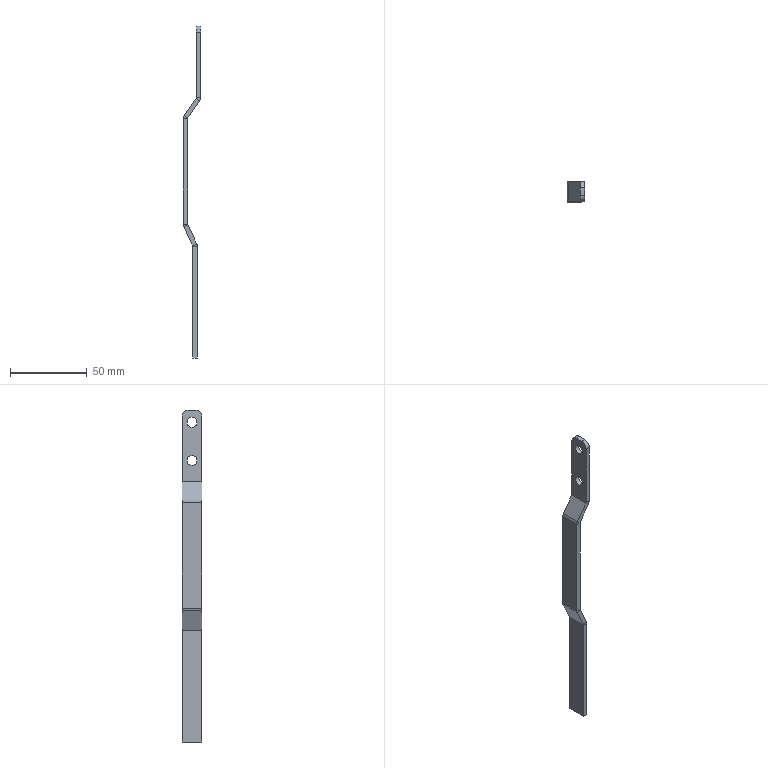Component | SolidWorks | GlassDoorAssembly-1_828LockAssembly-1_LowerPullRod-1 | 1 solid | 44 faces | volume 8395 mm3 | plane 30 | cylinder 14 | commonest cylinder face diameters 6.5 x4 7.473 x4 1.473 x4 8 x2